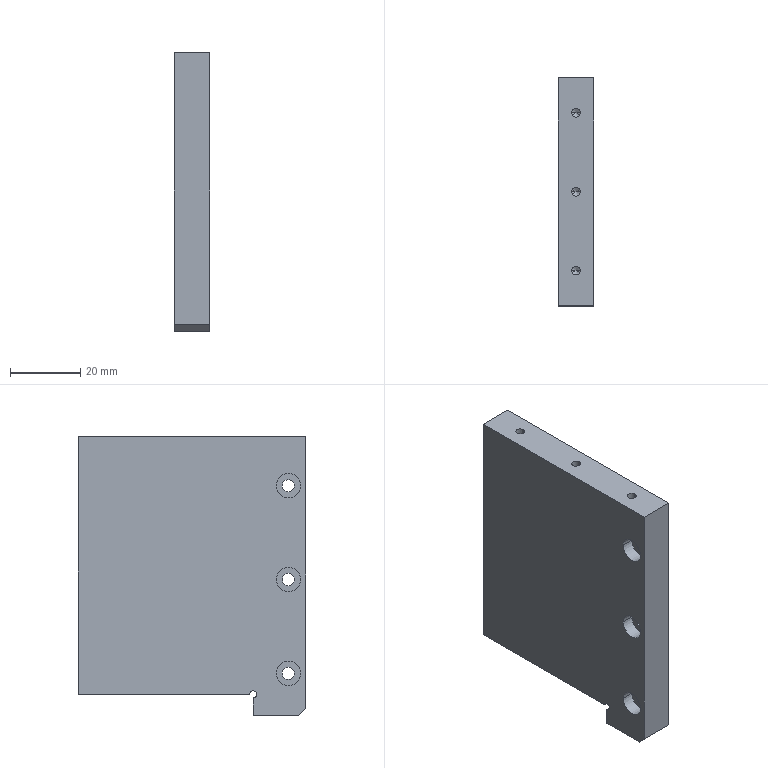Component | SolidWorks | 170423A4-SafetyPowerProbeFixingPlate2-1 | 1 solid | 62 faces | box 10 x 65 x 79.5 mm | volume 47436 mm3 | cylinder 33 | plane 15 | cone 14 | commonest cylinder face diameters 2.5 x14 7 x12 3.5 x6 2 x1
build123d program:
from build123d import *

# Parameters (mm, degrees)
SKETCH1_W                                       = 65
SKETCH1_H                                       = 73.5
BOSS_EXTRUDE1_DEPTH                             = 10
SKETCH2_W                                       = 15
SKETCH2_H                                       = 10
BOSS_EXTRUDE2_DEPTH                             = 6
SKETCH3_R                                       = 1
CUT_EXTRUDE1_DEPTH                              = 104.176
CHAMFER1_SIZE                                   = 2
M3_TAPPED_HOLE1_D                               = 2.5
M3_TAPPED_HOLE1_DEPTH                           = 8.5
M3_TAPPED_HOLE1_TIP                             = 0.7511
M3_TAPPED_HOLE2_D                               = 2.5
M3_TAPPED_HOLE2_DEPTH                           = 8.5
M3_TAPPED_HOLE2_TIP                             = 0.7511
M3_HEX_SOCKET_HEAD_CAP_SCREW_CBORE1_D           = 3.5
M3_HEX_SOCKET_HEAD_CAP_SCREW_CBORE1_CBORE_D     = 7
M3_HEX_SOCKET_HEAD_CAP_SCREW_CBORE1_CBORE_DEPTH = 3.5
CUT_EXTRUDE2_START                              = -3.5
SKETCH10_R                                      = 3.5
CUT_EXTRUDE2_DEPTH                              = 3.5
M3_TAPPED_HOLE3_D                               = 2.5
M3_TAPPED_HOLE3_DEPTH                           = 8.5
M3_TAPPED_HOLE3_TIP                             = 0.7511


with BuildPart() as part:
    # Sketch1 → Boss-Extrude1 (new body)
    with BuildSketch(Plane.XY):
        with Locations((32.5, 36.75)):
            Rectangle(SKETCH1_W, SKETCH1_H)
    extrude(amount=BOSS_EXTRUDE1_DEPTH)

    # Sketch2 → Boss-Extrude2 (add)
    with BuildSketch(Plane(origin=(0, 73.5, 0), x_dir=(1, 0, 0), z_dir=(0, 1, 0))):
        with Locations((7.5, -5)):
            Rectangle(SKETCH2_W, SKETCH2_H)
    extrude(amount=BOSS_EXTRUDE2_DEPTH)

    # Sketch3 → Cut-Extrude1 (cut, through all)
    with BuildSketch(Plane.XY.offset(10)):
        with Locations((15, 73.5)):
            Circle(SKETCH3_R)
    extrude(amount=-CUT_EXTRUDE1_DEPTH, mode=Mode.SUBTRACT)

    # Chamfer1
    chamfer1_edges = [part.edges().sort_by_distance(p)[0] for p in [
        (0, 79.5, 5),
    ]]
    chamfer(chamfer1_edges, length=CHAMFER1_SIZE)

    # M3 Tapped Hole1
    with Locations(Plane(origin=(0, 73.5, 0), x_dir=(1, 0, 0), z_dir=(0, 1, 0))):
        with Locations((23, -5), (57, -5)):
            Hole(M3_TAPPED_HOLE1_D / 2, depth=M3_TAPPED_HOLE1_DEPTH)
            with Locations((0, 0, -(M3_TAPPED_HOLE1_DEPTH + M3_TAPPED_HOLE1_TIP / 2))):  # 118° drill point
                Cone(0, M3_TAPPED_HOLE1_D / 2, M3_TAPPED_HOLE1_TIP, mode=Mode.SUBTRACT)

    # M3 Tapped Hole2
    with Locations(Plane(origin=(0, 0, 0), x_dir=(-1, 0, 0), z_dir=(0, -1, 0))):
        with Locations((-32.5, -5), (-10, -5), (-55, -5)):
            Hole(M3_TAPPED_HOLE2_D / 2, depth=M3_TAPPED_HOLE2_DEPTH)
            with Locations((0, 0, -(M3_TAPPED_HOLE2_DEPTH + M3_TAPPED_HOLE2_TIP / 2))):  # 118° drill point
                Cone(0, M3_TAPPED_HOLE2_D / 2, M3_TAPPED_HOLE2_TIP, mode=Mode.SUBTRACT)

    # M3 Hex Socket Head Cap Screw CBORE1 (through all)
    with Locations(Plane.XY.offset(10)):
        with Locations((5, 67.5), (5, 40.75), (5, 14)):
            CounterBoreHole(M3_HEX_SOCKET_HEAD_CAP_SCREW_CBORE1_D / 2, M3_HEX_SOCKET_HEAD_CAP_SCREW_CBORE1_CBORE_D / 2, M3_HEX_SOCKET_HEAD_CAP_SCREW_CBORE1_CBORE_DEPTH)

    # Sketch10 → Cut-Extrude2 (cut)
    with BuildSketch(Plane(origin=(0, 0, 0), x_dir=(-1, 0, 0), z_dir=(0, 0, -1)).offset(CUT_EXTRUDE2_START)):
        with Locations(Location((-5, 14, 0), (0, 0, 180))):
            Circle(SKETCH10_R)
        with Locations(Location((-5, 40.75, 0), (0, 0, 180))):
            Circle(SKETCH10_R)
        with Locations(Location((-5, 67.5, 0), (0, 0, 180))):
            Circle(SKETCH10_R)
    extrude(amount=CUT_EXTRUDE2_DEPTH, mode=Mode.SUBTRACT)

    # M3 Tapped Hole3
    with Locations(Plane(origin=(65, 0, 0), x_dir=(0, 0, -1), z_dir=(1, 0, 0))):
        with Locations((-5, 63.5), (-5, 12)):
            Hole(M3_TAPPED_HOLE3_D / 2, depth=M3_TAPPED_HOLE3_DEPTH)
            with Locations((0, 0, -(M3_TAPPED_HOLE3_DEPTH + M3_TAPPED_HOLE3_TIP / 2))):  # 118° drill point
                Cone(0, M3_TAPPED_HOLE3_D / 2, M3_TAPPED_HOLE3_TIP, mode=Mode.SUBTRACT)


solid = part.part

# Placed as in the assembly
solid = solid.moved(Location((-16.313, -25.611, -0.07379), (-90, -90, 0)))